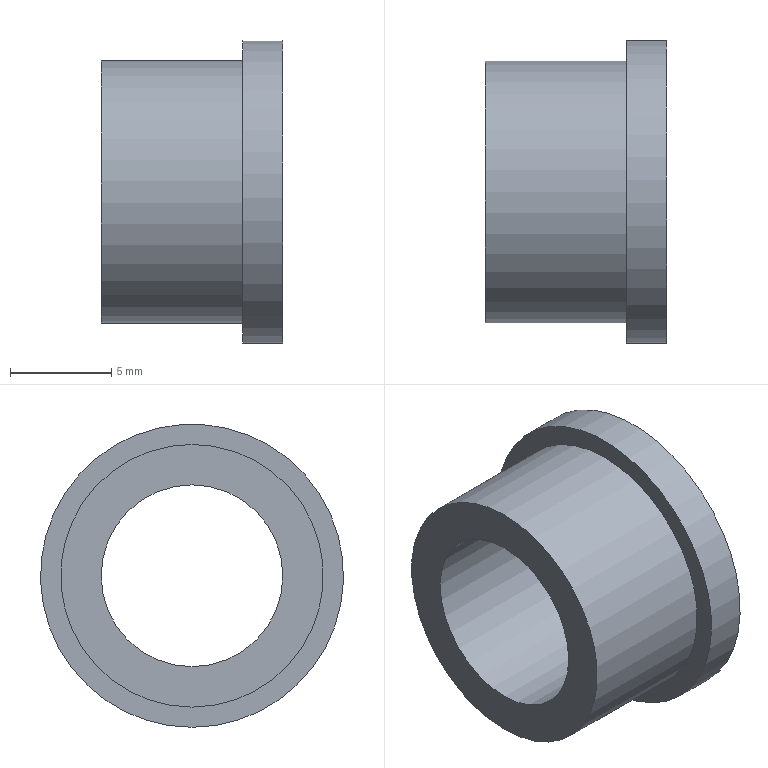Component | NX | LOCATING_BUSH_2 | 1 solid | 6 faces | box 9 x 15 x 15 mm | volume 710 mm3 | plane 3 | cylinder 3 | commonest cylinder face diameters 13 x1 15 x1 9 x1
STEP:
#1=CARTESIAN_POINT('',(0.,0.,0.));
#2=DIRECTION('',(0.,0.,1.));
#3=DIRECTION('',(1.,0.,0.));
#4=AXIS2_PLACEMENT_3D('',#1,#2,#3);
#5=CARTESIAN_POINT('',(-21.772,-17.527,-184.219));
#6=VERTEX_POINT('',#5);
#7=CARTESIAN_POINT('',(-21.772,-17.527,-188.719));
#8=DIRECTION('',(-1.,0.,0.));
#9=DIRECTION('',(0.,0.,1.));
#10=AXIS2_PLACEMENT_3D('',#7,#8,#9);
#11=CIRCLE('',#10,4.5);
#12=CARTESIAN_POINT('',(-21.772,-17.527,-188.719));
#13=DIRECTION('',(-1.,0.,0.));
#14=DIRECTION('',(0.,0.,1.));
#15=AXIS2_PLACEMENT_3D('',#12,#13,#14);
#16=PLANE('',#15);
#17=CARTESIAN_POINT('',(0.,0.));
#18=DIRECTION('',(1.,0.));
#19=AXIS2_PLACEMENT_2D('',#17,#18);
#20=CIRCLE('',#19,4.5);
#21=(GEOMETRIC_REPRESENTATION_CONTEXT(2)PARAMETRIC_REPRESENTATION_CONTEXT()REPRESENTATION_CONTEXT('',''));
#22=DEFINITIONAL_REPRESENTATION('',(#20),#21);
#23=PCURVE('',#16,#22);
#24=CARTESIAN_POINT('',(-12.772,-17.527,-188.719));
#25=DIRECTION('',(-1.,0.,0.));
#26=DIRECTION('',(0.,0.,1.));
#27=AXIS2_PLACEMENT_3D('',#24,#25,#26);
#28=CYLINDRICAL_SURFACE('',#27,4.5);
#29=CARTESIAN_POINT('',(0.,9.));
#30=DIRECTION('',(1.,0.));
#31=VECTOR('',#30,1.);
#32=LINE('',#29,#31);
#33=(GEOMETRIC_REPRESENTATION_CONTEXT(2)PARAMETRIC_REPRESENTATION_CONTEXT()REPRESENTATION_CONTEXT('',''));
#34=DEFINITIONAL_REPRESENTATION('',(#32),#33);
#35=PCURVE('',#28,#34);
#36=SURFACE_CURVE('',#11,(#23,#35),.PCURVE_S1.);
#37=EDGE_CURVE('',#6,#6,#36,.T.);
#38=ORIENTED_EDGE('',*,*,#37,.F.);
#39=EDGE_LOOP('',(#38));
#40=FACE_BOUND('',#39,.T.);
#41=CARTESIAN_POINT('',(-21.772,-17.527,-195.219));
#42=VERTEX_POINT('',#41);
#43=CARTESIAN_POINT('',(-21.772,-17.527,-188.719));
#44=DIRECTION('',(1.,0.,0.));
#45=DIRECTION('',(0.,0.,-1.));
#46=AXIS2_PLACEMENT_3D('',#43,#44,#45);
#47=CIRCLE('',#46,6.5);
#48=CARTESIAN_POINT('',(-6.5,0.));
#49=CARTESIAN_POINT('',(-6.5,11.258));
#50=CARTESIAN_POINT('',(3.25,5.629));
#51=CARTESIAN_POINT('',(13.,0.));
#52=CARTESIAN_POINT('',(3.25,-5.629));
#53=CARTESIAN_POINT('',(-6.5,-11.258));
#54=CARTESIAN_POINT('',(-6.5,0.));
#55=(BOUNDED_CURVE()B_SPLINE_CURVE(2,(#48,#49,#50,#51,#52,#53,#54),.UNSPECIFIED.,.T.,.F.)B_SPLINE_CURVE_WITH_KNOTS((1,2,2,2,2,1),(-2.094,0.,2.094,4.189,6.283,8.378),.UNSPECIFIED.)CURVE()GEOMETRIC_REPRESENTATION_ITEM()RATIONAL_B_SPLINE_CURVE((1.,0.5,1.,0.5,1.,0.5,1.))REPRESENTATION_ITEM(''));
#56=(GEOMETRIC_REPRESENTATION_CONTEXT(2)PARAMETRIC_REPRESENTATION_CONTEXT()REPRESENTATION_CONTEXT('',''));
#57=DEFINITIONAL_REPRESENTATION('',(#55),#56);
#58=PCURVE('',#16,#57);
#59=CARTESIAN_POINT('',(-21.772,-17.527,-188.719));
#60=DIRECTION('',(1.,0.,0.));
#61=DIRECTION('',(0.,0.,-1.));
#62=AXIS2_PLACEMENT_3D('',#59,#60,#61);
#63=CYLINDRICAL_SURFACE('',#62,6.5);
#64=CARTESIAN_POINT('',(0.,0.));
#65=DIRECTION('',(1.,0.));
#66=VECTOR('',#65,1.);
#67=LINE('',#64,#66);
#68=(GEOMETRIC_REPRESENTATION_CONTEXT(2)PARAMETRIC_REPRESENTATION_CONTEXT()REPRESENTATION_CONTEXT('',''));
#69=DEFINITIONAL_REPRESENTATION('',(#67),#68);
#70=PCURVE('',#63,#69);
#71=SURFACE_CURVE('',#47,(#58,#70),.PCURVE_S1.);
#72=EDGE_CURVE('',#42,#42,#71,.T.);
#73=ORIENTED_EDGE('',*,*,#72,.F.);
#74=EDGE_LOOP('',(#73));
#75=FACE_BOUND('',#74,.T.);
#76=ADVANCED_FACE('',(#40,#75),#16,.T.);
#77=CARTESIAN_POINT('',(-14.772,-17.527,-195.219));
#78=VERTEX_POINT('',#77);
#79=CARTESIAN_POINT('',(-14.772,-17.527,-182.219));
#80=VERTEX_POINT('',#79);
#81=CARTESIAN_POINT('',(-14.772,-17.527,-188.719));
#82=DIRECTION('',(1.,0.,0.));
#83=DIRECTION('',(0.,0.,1.));
#84=AXIS2_PLACEMENT_3D('',#81,#82,#83);
#85=CIRCLE('',#84,6.5);
#86=CARTESIAN_POINT('',(-3.142,7.));
#87=DIRECTION('',(1.,0.));
#88=VECTOR('',#87,1.);
#89=LINE('',#86,#88);
#90=(GEOMETRIC_REPRESENTATION_CONTEXT(2)PARAMETRIC_REPRESENTATION_CONTEXT()REPRESENTATION_CONTEXT('',''));
#91=DEFINITIONAL_REPRESENTATION('',(#89),#90);
#92=PCURVE('',#63,#91);
#93=CARTESIAN_POINT('',(-14.772,-17.527,-188.719));
#94=DIRECTION('',(-1.,0.,0.));
#95=DIRECTION('',(0.,0.,1.));
#96=AXIS2_PLACEMENT_3D('',#93,#94,#95);
#97=PLANE('',#96);
#98=CARTESIAN_POINT('',(6.5,0.));
#99=CARTESIAN_POINT('',(6.5,-11.258));
#100=CARTESIAN_POINT('',(-3.25,-5.629));
#101=CARTESIAN_POINT('',(-13.,-0.));
#102=CARTESIAN_POINT('',(-3.25,5.629));
#103=CARTESIAN_POINT('',(6.5,11.258));
#104=CARTESIAN_POINT('',(6.5,0.));
#105=(BOUNDED_CURVE()B_SPLINE_CURVE(2,(#98,#99,#100,#101,#102,#103,#104),.UNSPECIFIED.,.T.,.F.)B_SPLINE_CURVE_WITH_KNOTS((1,2,2,2,2,1),(-2.094,0.,2.094,4.189,6.283,8.378),.UNSPECIFIED.)CURVE()GEOMETRIC_REPRESENTATION_ITEM()RATIONAL_B_SPLINE_CURVE((1.,0.5,1.,0.5,1.,0.5,1.))REPRESENTATION_ITEM(''));
#106=(GEOMETRIC_REPRESENTATION_CONTEXT(2)PARAMETRIC_REPRESENTATION_CONTEXT()REPRESENTATION_CONTEXT('',''));
#107=DEFINITIONAL_REPRESENTATION('',(#105),#106);
#108=PCURVE('',#97,#107);
#109=SURFACE_CURVE('',#85,(#92,#108),.PCURVE_S1.);
#110=EDGE_CURVE('',#78,#80,#109,.T.);
#111=ORIENTED_EDGE('',*,*,#110,.F.);
#112=CARTESIAN_POINT('',(-21.772,-17.527,-195.219));
#113=CARTESIAN_POINT('',(-14.772,-17.527,-195.219));
#114=B_SPLINE_CURVE_WITH_KNOTS('',1,(#112,#113),.UNSPECIFIED.,.F.,.F.,(2,2),(0.,7.),.PIECEWISE_BEZIER_KNOTS.);
#115=CARTESIAN_POINT('',(0.,0.));
#116=DIRECTION('',(0.,1.));
#117=VECTOR('',#116,1.);
#118=LINE('',#115,#117);
#119=(GEOMETRIC_REPRESENTATION_CONTEXT(2)PARAMETRIC_REPRESENTATION_CONTEXT()REPRESENTATION_CONTEXT('',''));
#120=DEFINITIONAL_REPRESENTATION('',(#118),#119);
#121=PCURVE('',#63,#120);
#122=CARTESIAN_POINT('',(6.283,0.));
#123=DIRECTION('',(0.,1.));
#124=VECTOR('',#123,1.);
#125=LINE('',#122,#124);
#126=(GEOMETRIC_REPRESENTATION_CONTEXT(2)PARAMETRIC_REPRESENTATION_CONTEXT()REPRESENTATION_CONTEXT('',''));
#127=DEFINITIONAL_REPRESENTATION('',(#125),#126);
#128=PCURVE('',#63,#127);
#129=SEAM_CURVE('',#114,(#121,#128),.PCURVE_S1.);
#130=EDGE_CURVE('',#42,#78,#129,.T.);
#131=ORIENTED_EDGE('',*,*,#130,.F.);
#132=ORIENTED_EDGE('',*,*,#72,.T.);
#133=ORIENTED_EDGE('',*,*,#130,.T.);
#134=CARTESIAN_POINT('',(-14.772,-17.527,-188.719));
#135=DIRECTION('',(1.,0.,0.));
#136=DIRECTION('',(0.,0.,1.));
#137=AXIS2_PLACEMENT_3D('',#134,#135,#136);
#138=CIRCLE('',#137,6.5);
#139=CARTESIAN_POINT('',(3.142,7.));
#140=DIRECTION('',(1.,0.));
#141=VECTOR('',#140,1.);
#142=LINE('',#139,#141);
#143=(GEOMETRIC_REPRESENTATION_CONTEXT(2)PARAMETRIC_REPRESENTATION_CONTEXT()REPRESENTATION_CONTEXT('',''));
#144=DEFINITIONAL_REPRESENTATION('',(#142),#143);
#145=PCURVE('',#63,#144);
#146=CARTESIAN_POINT('',(6.5,0.));
#147=CARTESIAN_POINT('',(6.5,-11.258));
#148=CARTESIAN_POINT('',(-3.25,-5.629));
#149=CARTESIAN_POINT('',(-13.,-0.));
#150=CARTESIAN_POINT('',(-3.25,5.629));
#151=CARTESIAN_POINT('',(6.5,11.258));
#152=CARTESIAN_POINT('',(6.5,0.));
#153=(BOUNDED_CURVE()B_SPLINE_CURVE(2,(#146,#147,#148,#149,#150,#151,#152),.UNSPECIFIED.,.T.,.F.)B_SPLINE_CURVE_WITH_KNOTS((1,2,2,2,2,1),(-2.094,0.,2.094,4.189,6.283,8.378),.UNSPECIFIED.)CURVE()GEOMETRIC_REPRESENTATION_ITEM()RATIONAL_B_SPLINE_CURVE((1.,0.5,1.,0.5,1.,0.5,1.))REPRESENTATION_ITEM(''));
#154=(GEOMETRIC_REPRESENTATION_CONTEXT(2)PARAMETRIC_REPRESENTATION_CONTEXT()REPRESENTATION_CONTEXT('',''));
#155=DEFINITIONAL_REPRESENTATION('',(#153),#154);
#156=PCURVE('',#97,#155);
#157=SURFACE_CURVE('',#138,(#145,#156),.PCURVE_S1.);
#158=EDGE_CURVE('',#80,#78,#157,.T.);
#159=ORIENTED_EDGE('',*,*,#158,.F.);
#160=EDGE_LOOP('',(#111,#131,#132,#133,#159));
#161=FACE_BOUND('',#160,.T.);
#162=ADVANCED_FACE('',(#161),#63,.T.);
#163=CARTESIAN_POINT('',(-12.772,-17.527,-184.219));
#164=VERTEX_POINT('',#163);
#165=CARTESIAN_POINT('',(-12.772,-17.527,-188.719));
#166=DIRECTION('',(-1.,0.,0.));
#167=DIRECTION('',(0.,0.,1.));
#168=AXIS2_PLACEMENT_3D('',#165,#166,#167);
#169=CIRCLE('',#168,4.5);
#170=CARTESIAN_POINT('',(-12.772,-17.527,-188.719));
#171=DIRECTION('',(1.,0.,0.));
#172=DIRECTION('',(0.,0.,-1.));
#173=AXIS2_PLACEMENT_3D('',#170,#171,#172);
#174=PLANE('',#173);
#175=CARTESIAN_POINT('',(-4.5,0.));
#176=CARTESIAN_POINT('',(-4.5,7.794));
#177=CARTESIAN_POINT('',(2.25,3.897));
#178=CARTESIAN_POINT('',(9.,0.));
#179=CARTESIAN_POINT('',(2.25,-3.897));
#180=CARTESIAN_POINT('',(-4.5,-7.794));
#181=CARTESIAN_POINT('',(-4.5,0.));
#182=(BOUNDED_CURVE()B_SPLINE_CURVE(2,(#175,#176,#177,#178,#179,#180,#181),.UNSPECIFIED.,.T.,.F.)B_SPLINE_CURVE_WITH_KNOTS((1,2,2,2,2,1),(-2.094,0.,2.094,4.189,6.283,8.378),.UNSPECIFIED.)CURVE()GEOMETRIC_REPRESENTATION_ITEM()RATIONAL_B_SPLINE_CURVE((1.,0.5,1.,0.5,1.,0.5,1.))REPRESENTATION_ITEM(''));
#183=(GEOMETRIC_REPRESENTATION_CONTEXT(2)PARAMETRIC_REPRESENTATION_CONTEXT()REPRESENTATION_CONTEXT('',''));
#184=DEFINITIONAL_REPRESENTATION('',(#182),#183);
#185=PCURVE('',#174,#184);
#186=CARTESIAN_POINT('',(0.,0.));
#187=DIRECTION('',(1.,0.));
#188=VECTOR('',#187,1.);
#189=LINE('',#186,#188);
#190=(GEOMETRIC_REPRESENTATION_CONTEXT(2)PARAMETRIC_REPRESENTATION_CONTEXT()REPRESENTATION_CONTEXT('',''));
#191=DEFINITIONAL_REPRESENTATION('',(#189),#190);
#192=PCURVE('',#28,#191);
#193=SURFACE_CURVE('',#169,(#185,#192),.PCURVE_S1.);
#194=EDGE_CURVE('',#164,#164,#193,.T.);
#195=ORIENTED_EDGE('',*,*,#194,.T.);
#196=EDGE_LOOP('',(#195));
#197=FACE_BOUND('',#196,.T.);
#198=CARTESIAN_POINT('',(-12.772,-17.527,-196.219));
#199=VERTEX_POINT('',#198);
#200=CARTESIAN_POINT('',(-12.772,-17.527,-188.719));
#201=DIRECTION('',(-1.,0.,0.));
#202=DIRECTION('',(0.,0.,-1.));
#203=AXIS2_PLACEMENT_3D('',#200,#201,#202);
#204=CIRCLE('',#203,7.5);
#205=CARTESIAN_POINT('',(7.5,0.));
#206=CARTESIAN_POINT('',(7.5,-12.99));
#207=CARTESIAN_POINT('',(-3.75,-6.495));
#208=CARTESIAN_POINT('',(-15.,-0.));
#209=CARTESIAN_POINT('',(-3.75,6.495));
#210=CARTESIAN_POINT('',(7.5,12.99));
#211=CARTESIAN_POINT('',(7.5,0.));
#212=(BOUNDED_CURVE()B_SPLINE_CURVE(2,(#205,#206,#207,#208,#209,#210,#211),.UNSPECIFIED.,.T.,.F.)B_SPLINE_CURVE_WITH_KNOTS((1,2,2,2,2,1),(-2.094,0.,2.094,4.189,6.283,8.378),.UNSPECIFIED.)CURVE()GEOMETRIC_REPRESENTATION_ITEM()RATIONAL_B_SPLINE_CURVE((1.,0.5,1.,0.5,1.,0.5,1.))REPRESENTATION_ITEM(''));
#213=(GEOMETRIC_REPRESENTATION_CONTEXT(2)PARAMETRIC_REPRESENTATION_CONTEXT()REPRESENTATION_CONTEXT('',''));
#214=DEFINITIONAL_REPRESENTATION('',(#212),#213);
#215=PCURVE('',#174,#214);
#216=CARTESIAN_POINT('',(-14.772,-17.527,-188.719));
#217=DIRECTION('',(1.,0.,0.));
#218=DIRECTION('',(0.,0.,-1.));
#219=AXIS2_PLACEMENT_3D('',#216,#217,#218);
#220=CYLINDRICAL_SURFACE('',#219,7.5);
#221=CARTESIAN_POINT('',(6.283,2.));
#222=DIRECTION('',(-1.,0.));
#223=VECTOR('',#222,1.);
#224=LINE('',#221,#223);
#225=(GEOMETRIC_REPRESENTATION_CONTEXT(2)PARAMETRIC_REPRESENTATION_CONTEXT()REPRESENTATION_CONTEXT('',''));
#226=DEFINITIONAL_REPRESENTATION('',(#224),#225);
#227=PCURVE('',#220,#226);
#228=SURFACE_CURVE('',#204,(#215,#227),.PCURVE_S1.);
#229=EDGE_CURVE('',#199,#199,#228,.T.);
#230=ORIENTED_EDGE('',*,*,#229,.F.);
#231=EDGE_LOOP('',(#230));
#232=FACE_BOUND('',#231,.T.);
#233=ADVANCED_FACE('',(#197,#232),#174,.T.);
#234=ORIENTED_EDGE('',*,*,#158,.T.);
#235=ORIENTED_EDGE('',*,*,#110,.T.);
#236=EDGE_LOOP('',(#234,#235));
#237=FACE_BOUND('',#236,.T.);
#238=CARTESIAN_POINT('',(-14.772,-17.527,-196.219));
#239=VERTEX_POINT('',#238);
#240=CARTESIAN_POINT('',(-14.772,-17.527,-188.719));
#241=DIRECTION('',(1.,0.,0.));
#242=DIRECTION('',(0.,0.,-1.));
#243=AXIS2_PLACEMENT_3D('',#240,#241,#242);
#244=CIRCLE('',#243,7.5);
#245=CARTESIAN_POINT('',(-7.5,0.));
#246=CARTESIAN_POINT('',(-7.5,12.99));
#247=CARTESIAN_POINT('',(3.75,6.495));
#248=CARTESIAN_POINT('',(15.,0.));
#249=CARTESIAN_POINT('',(3.75,-6.495));
#250=CARTESIAN_POINT('',(-7.5,-12.99));
#251=CARTESIAN_POINT('',(-7.5,0.));
#252=(BOUNDED_CURVE()B_SPLINE_CURVE(2,(#245,#246,#247,#248,#249,#250,#251),.UNSPECIFIED.,.T.,.F.)B_SPLINE_CURVE_WITH_KNOTS((1,2,2,2,2,1),(-2.094,0.,2.094,4.189,6.283,8.378),.UNSPECIFIED.)CURVE()GEOMETRIC_REPRESENTATION_ITEM()RATIONAL_B_SPLINE_CURVE((1.,0.5,1.,0.5,1.,0.5,1.))REPRESENTATION_ITEM(''));
#253=(GEOMETRIC_REPRESENTATION_CONTEXT(2)PARAMETRIC_REPRESENTATION_CONTEXT()REPRESENTATION_CONTEXT('',''));
#254=DEFINITIONAL_REPRESENTATION('',(#252),#253);
#255=PCURVE('',#97,#254);
#256=CARTESIAN_POINT('',(0.,0.));
#257=DIRECTION('',(1.,0.));
#258=VECTOR('',#257,1.);
#259=LINE('',#256,#258);
#260=(GEOMETRIC_REPRESENTATION_CONTEXT(2)PARAMETRIC_REPRESENTATION_CONTEXT()REPRESENTATION_CONTEXT('',''));
#261=DEFINITIONAL_REPRESENTATION('',(#259),#260);
#262=PCURVE('',#220,#261);
#263=SURFACE_CURVE('',#244,(#255,#262),.PCURVE_S1.);
#264=EDGE_CURVE('',#239,#239,#263,.T.);
#265=ORIENTED_EDGE('',*,*,#264,.F.);
#266=EDGE_LOOP('',(#265));
#267=FACE_BOUND('',#266,.T.);
#268=ADVANCED_FACE('',(#237,#267),#97,.T.);
#269=ORIENTED_EDGE('',*,*,#229,.T.);
#270=CARTESIAN_POINT('',(-14.772,-17.527,-196.219));
#271=CARTESIAN_POINT('',(-12.772,-17.527,-196.219));
#272=B_SPLINE_CURVE_WITH_KNOTS('',1,(#270,#271),.UNSPECIFIED.,.F.,.F.,(2,2),(0.,2.),.PIECEWISE_BEZIER_KNOTS.);
#273=CARTESIAN_POINT('',(0.,0.));
#274=DIRECTION('',(0.,1.));
#275=VECTOR('',#274,1.);
#276=LINE('',#273,#275);
#277=(GEOMETRIC_REPRESENTATION_CONTEXT(2)PARAMETRIC_REPRESENTATION_CONTEXT()REPRESENTATION_CONTEXT('',''));
#278=DEFINITIONAL_REPRESENTATION('',(#276),#277);
#279=PCURVE('',#220,#278);
#280=CARTESIAN_POINT('',(6.283,0.));
#281=DIRECTION('',(0.,1.));
#282=VECTOR('',#281,1.);
#283=LINE('',#280,#282);
#284=(GEOMETRIC_REPRESENTATION_CONTEXT(2)PARAMETRIC_REPRESENTATION_CONTEXT()REPRESENTATION_CONTEXT('',''));
#285=DEFINITIONAL_REPRESENTATION('',(#283),#284);
#286=PCURVE('',#220,#285);
#287=SEAM_CURVE('',#272,(#279,#286),.PCURVE_S1.);
#288=EDGE_CURVE('',#239,#199,#287,.T.);
#289=ORIENTED_EDGE('',*,*,#288,.F.);
#290=ORIENTED_EDGE('',*,*,#264,.T.);
#291=ORIENTED_EDGE('',*,*,#288,.T.);
#292=EDGE_LOOP('',(#269,#289,#290,#291));
#293=FACE_BOUND('',#292,.T.);
#294=ADVANCED_FACE('',(#293),#220,.T.);
#295=ORIENTED_EDGE('',*,*,#37,.F.);
#296=CARTESIAN_POINT('',(-12.772,-17.527,-184.219));
#297=CARTESIAN_POINT('',(-21.772,-17.527,-184.219));
#298=B_SPLINE_CURVE_WITH_KNOTS('',1,(#296,#297),.UNSPECIFIED.,.F.,.F.,(2,2),(0.,9.),.PIECEWISE_BEZIER_KNOTS.);
#299=CARTESIAN_POINT('',(0.,0.));
#300=DIRECTION('',(0.,1.));
#301=VECTOR('',#300,1.);
#302=LINE('',#299,#301);
#303=(GEOMETRIC_REPRESENTATION_CONTEXT(2)PARAMETRIC_REPRESENTATION_CONTEXT()REPRESENTATION_CONTEXT('',''));
#304=DEFINITIONAL_REPRESENTATION('',(#302),#303);
#305=PCURVE('',#28,#304);
#306=CARTESIAN_POINT('',(6.283,0.));
#307=DIRECTION('',(0.,1.));
#308=VECTOR('',#307,1.);
#309=LINE('',#306,#308);
#310=(GEOMETRIC_REPRESENTATION_CONTEXT(2)PARAMETRIC_REPRESENTATION_CONTEXT()REPRESENTATION_CONTEXT('',''));
#311=DEFINITIONAL_REPRESENTATION('',(#309),#310);
#312=PCURVE('',#28,#311);
#313=SEAM_CURVE('',#298,(#305,#312),.PCURVE_S1.);
#314=EDGE_CURVE('',#164,#6,#313,.T.);
#315=ORIENTED_EDGE('',*,*,#314,.F.);
#316=ORIENTED_EDGE('',*,*,#194,.T.);
#317=ORIENTED_EDGE('',*,*,#314,.T.);
#318=EDGE_LOOP('',(#295,#315,#316,#317));
#319=FACE_BOUND('',#318,.F.);
#320=ADVANCED_FACE('',(#319),#28,.F.);
#321=CLOSED_SHELL('',(#76,#162,#233,#268,#294,#320));
#322=MANIFOLD_SOLID_BREP('',#321);
#323=(LENGTH_UNIT()NAMED_UNIT(*)SI_UNIT(.MILLI.,.METRE.));
#324=UNCERTAINTY_MEASURE_WITH_UNIT(LENGTH_MEASURE(0.000005),#323,'','');
#325=(NAMED_UNIT(*)PLANE_ANGLE_UNIT()SI_UNIT($,.RADIAN.));
#326=(NAMED_UNIT(*)SI_UNIT($,.STERADIAN.)SOLID_ANGLE_UNIT());
#327=(GEOMETRIC_REPRESENTATION_CONTEXT(3)GLOBAL_UNCERTAINTY_ASSIGNED_CONTEXT((#324))GLOBAL_UNIT_ASSIGNED_CONTEXT((#323,#325,#326))REPRESENTATION_CONTEXT('',''));
#328=ADVANCED_BREP_SHAPE_REPRESENTATION('',(#4,#322),#327);